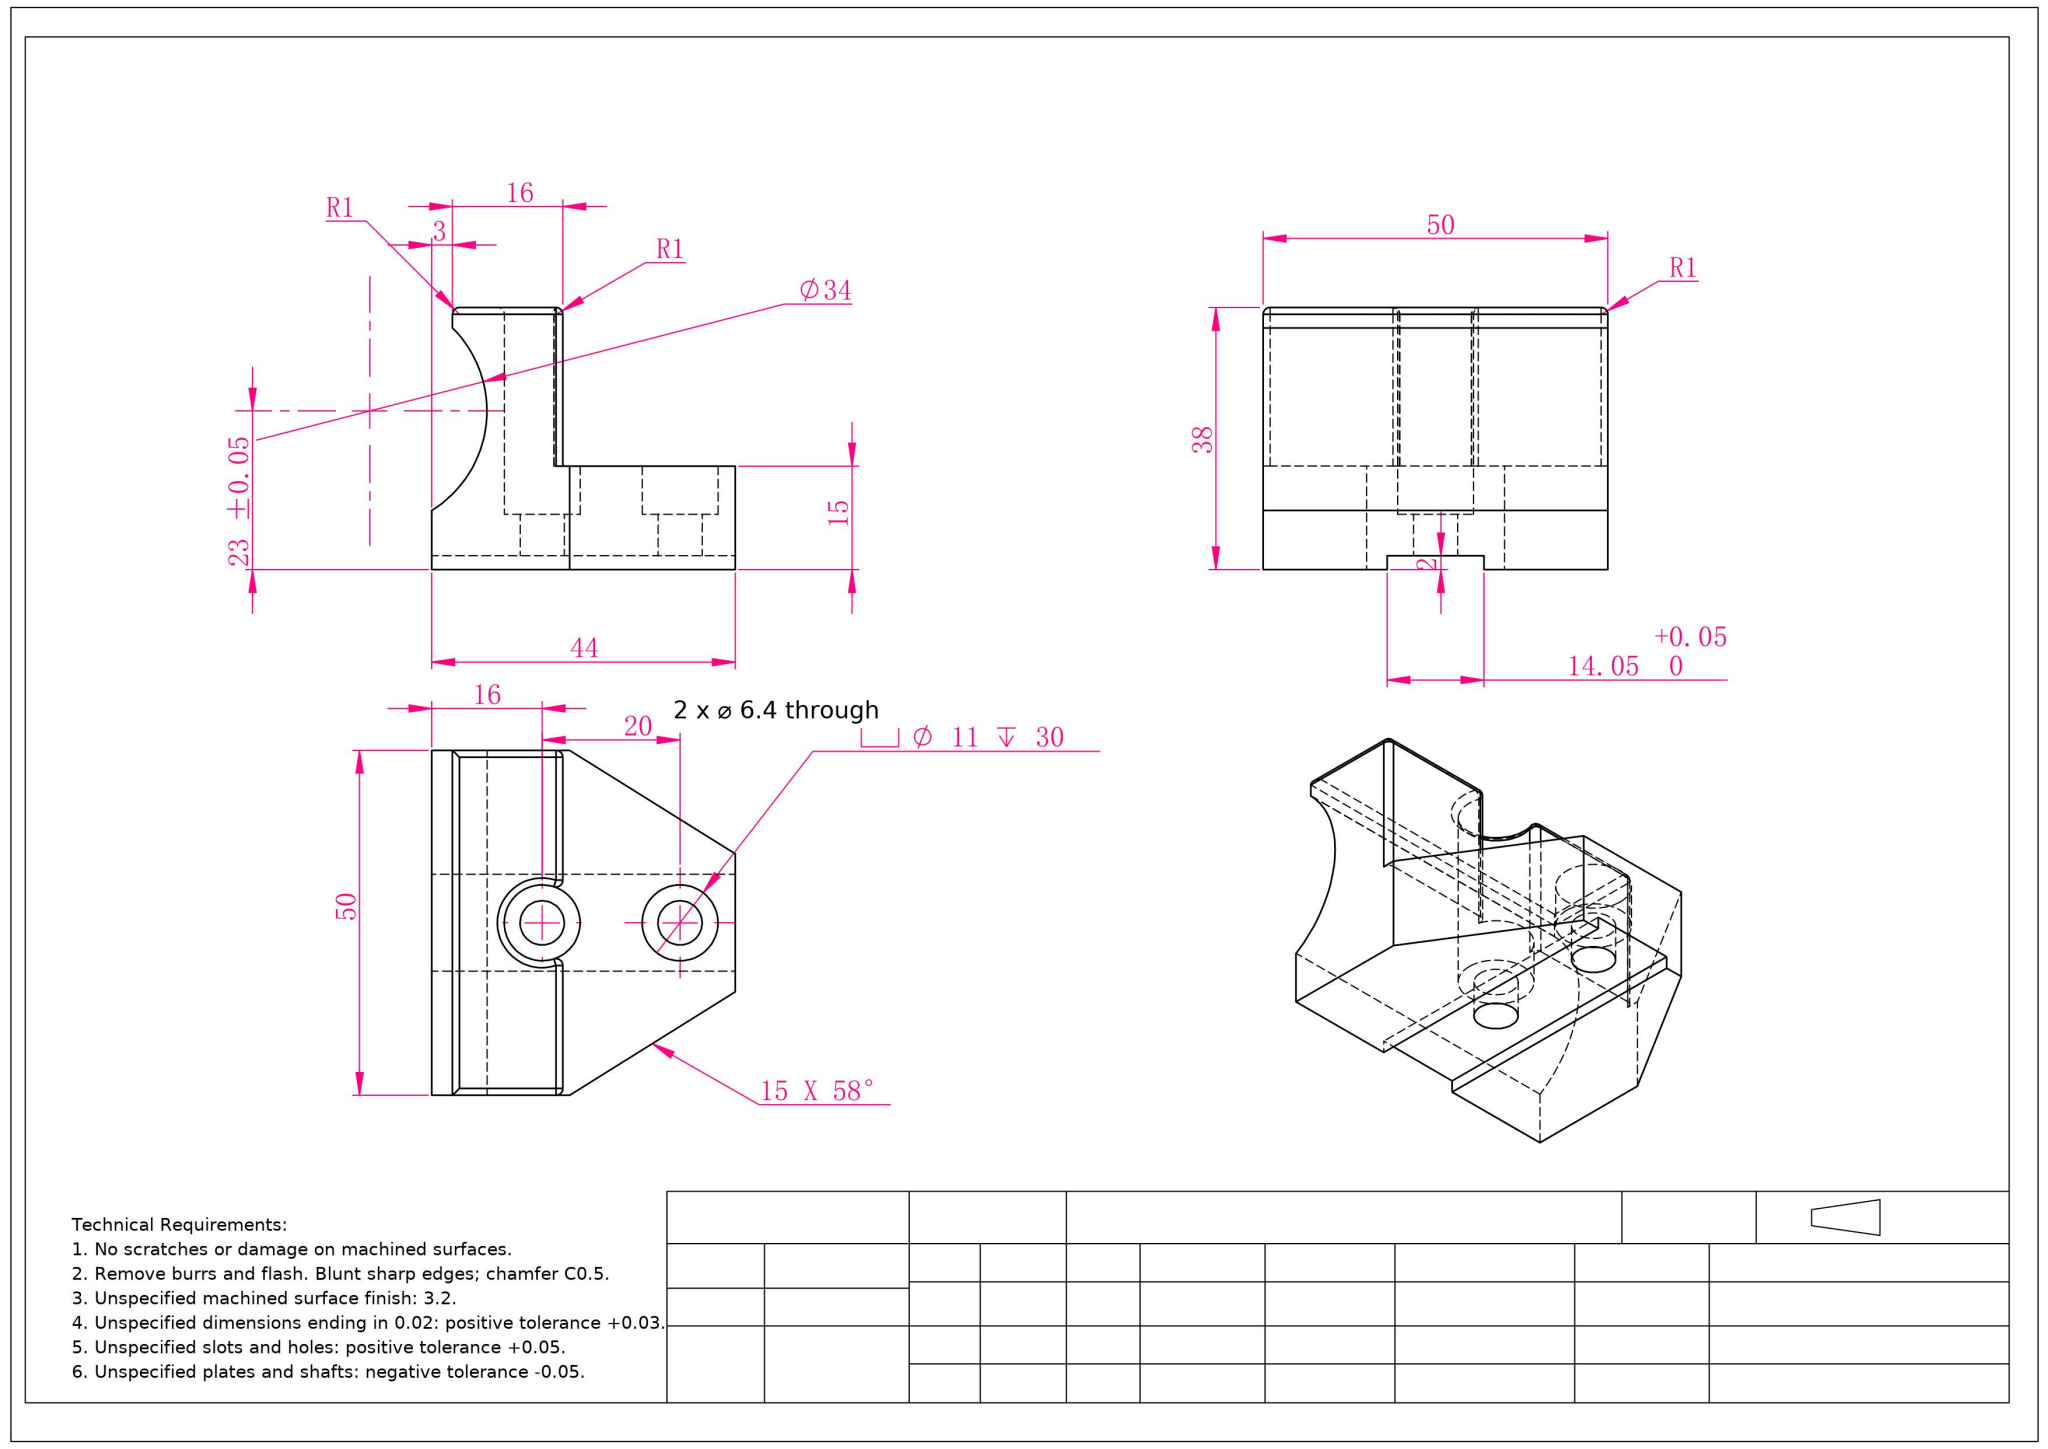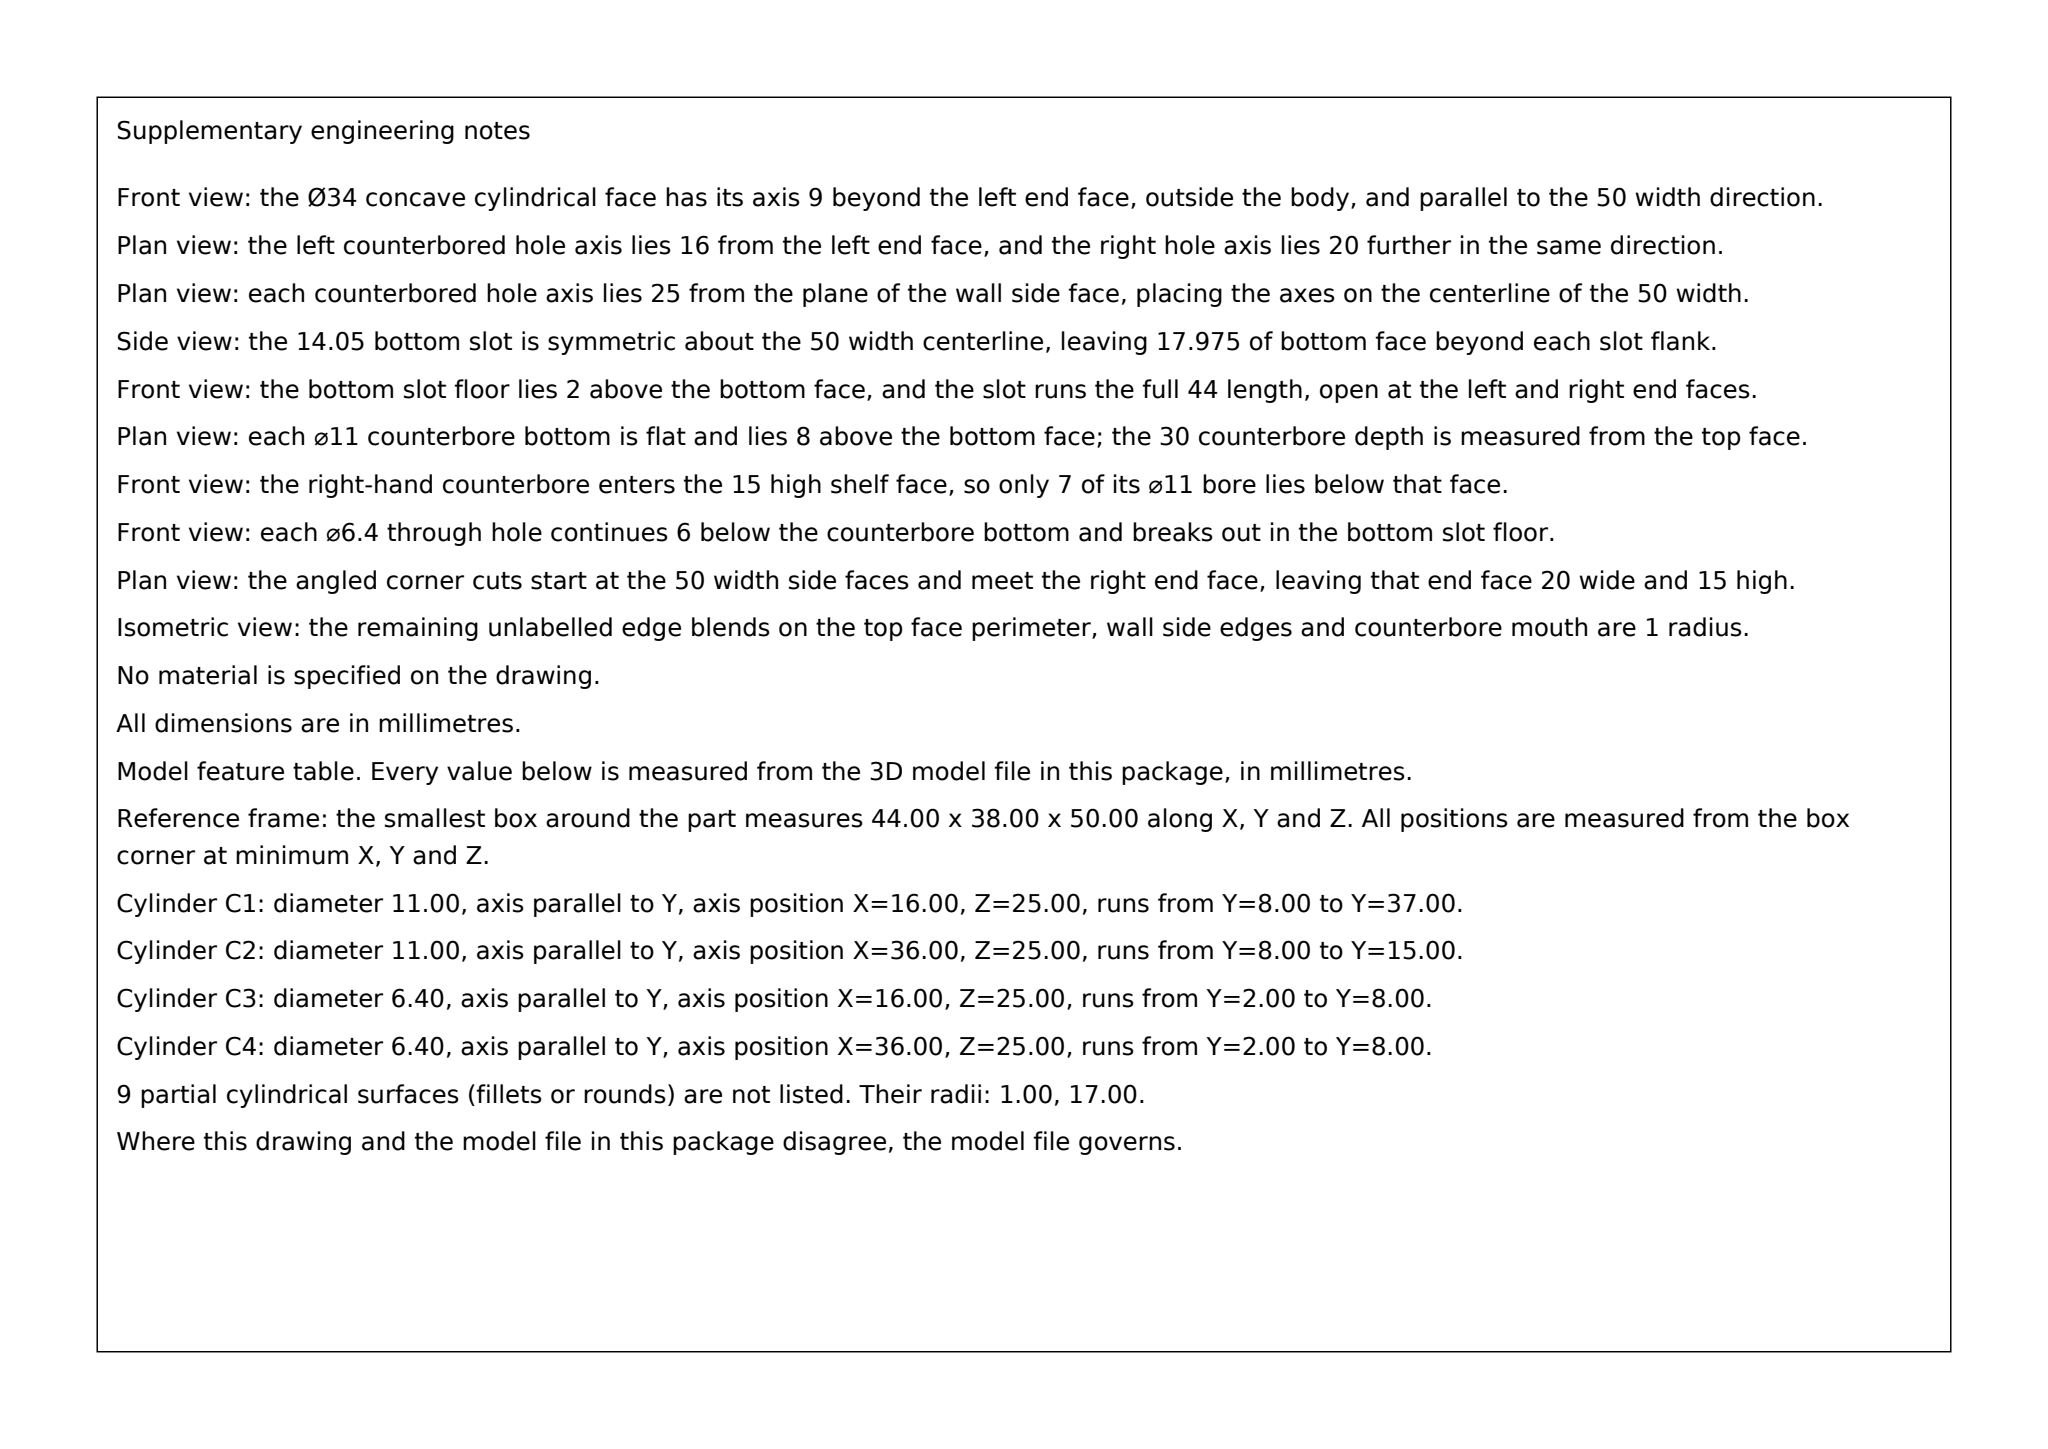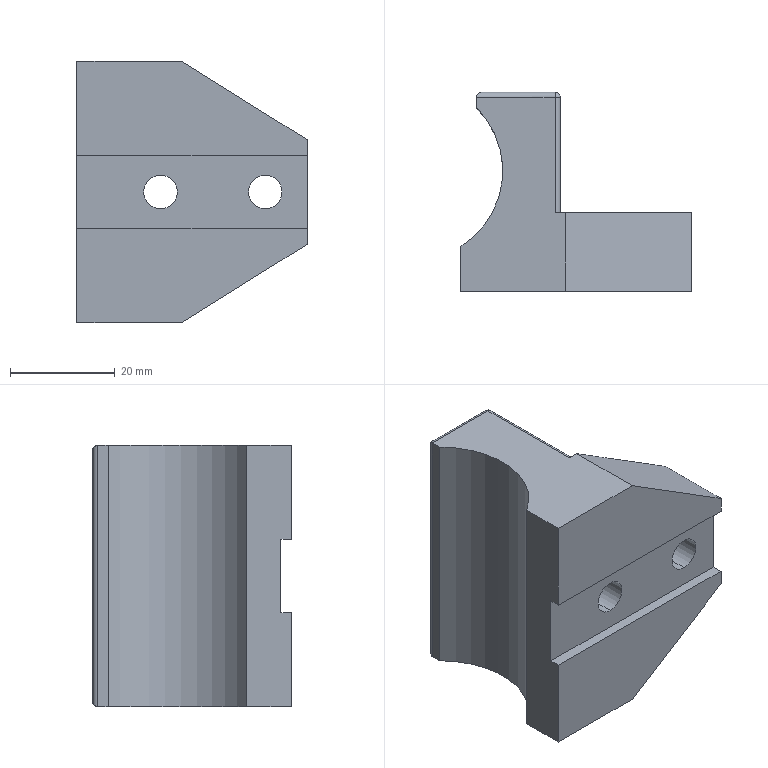Part | SolidWorks | mm | 1 solid | 44 faces | box 44 x 38 x 50 mm | volume 36222 mm3 | cylinder 19 | plane 18 | sphere 4 | torus 3 | commonest cylinder face diameters 2 x10 11 x4 6.4 x4 34 x1
Drawing notes:
3 & 16 WALLS 50 DEEP; TOP NOTCH 14.36 W CL ON 50 CL | from the solid: R1 edge cyl at (4,37) axis z len 50; top edge cyls at (18,37) len 17.82, vert R1 at z=18.82 & 31.18 -> gap 17.82-32.18 (14.36) centred on z=25
Ø34 CUT-OUT CL 9 OUTSIDE LH FACE, 23±0.05 UP FROM BASE | from the solid: cyl dia34 axis z at (x=-9, y=23); bbox x-min face x=0, base y=0
BOT SLOT 14.05 +0.05/0 W x 2 DP, 17.98 FROM FRONT 50 FACE | from the solid: z planes 17.98 & 32.03 (14.05 apart); y plane 2.0 = slot depth from y=0
2X Ø6.4 CBORE: 1ST CL 16 FROM LH FACE, 20 CTC, ON 50 CL | from the solid: dia6.4 axes y at x=16 and x=36, both z=25 (=50/2); spacing 20
NOTCH IN WALL BACK FACE: 14.36 W x 2 DP, 23 DOWN FROM TOP TO BASE | from the solid: R1 vert fillets at x=18, z=18.82/31.18 (len 22, y=15..37) => slot 17.82-32.18 (14.36 W, CL 25); fillet tangent x=17 vs back face x=19 (plane x=19 count 2) => 2 deep; wall y=15..38 => 23 from top face
HOLE AT 20 CTC: C'BORE Ø11 DP 7 FROM 15 BASE TOP FACE | from the solid: cylinder [11.0,"y",[36,null,25],7] vs [11.0,"y",[16,null,25],29]; base top plane y=15
build123d program:
from build123d import *
from OCP.BRepFilletAPI import BRepFilletAPI_MakeChamfer

# Parameters (mm, degrees)
BOSS_EXTRUDE1_DEPTH                             = 25
SKETCH2_W                                       = 45
SKETCH2_H                                       = 14.05
CUT_EXTRUDE1_DEPTH                              = 2
M6_HEX_SOCKET_HEAD_CAP_SCREW_CBORE1_D           = 6.4
M6_HEX_SOCKET_HEAD_CAP_SCREW_CBORE1_CBORE_D     = 11
M6_HEX_SOCKET_HEAD_CAP_SCREW_CBORE1_CBORE_DEPTH = 30
SKETCH6_W                                       = 25
SKETCH6_H                                       = 23
CUT_EXTRUDE3_DEPTH                              = 67.71
CUT_EXTRUDE4_DEPTH                              = 67.71
CHAMFER1_SIZE                                   = 15
CHAMFER1_SIZE2                                  = 24.005
FILLET1_R                                       = 1


with BuildPart() as part:
    # Sketch1 → Boss-Extrude1 (new, symmetric)
    with BuildSketch(Plane.XY):
        with BuildLine():
            Line((-22.5, 8), (-22.5, 0))
            Line((-22.5, 0), (22.5, 0))
            Line((22.5, 0), (22.5, 38))
            Line((22.5, 38), (-22.5, 38))
            ThreePointArc((-22.5, 38), (-15.923, 31.746), (-13.5, 23))
            ThreePointArc((-13.5, 23), (-15.923, 14.254), (-22.5, 8))
        make_face()
    extrude(amount=BOSS_EXTRUDE1_DEPTH, both=True)

    # Sketch2 → Cut-Extrude1 (cut)
    with BuildSketch(Plane.XZ):
        Rectangle(SKETCH2_W, SKETCH2_H)
    extrude(amount=-CUT_EXTRUDE1_DEPTH, mode=Mode.SUBTRACT)

    # M6 Hex Socket Head Cap Screw CBORE1 (through all)
    with Locations(Plane(origin=(0, 38, 0), x_dir=(1, 0, 0), z_dir=(0, 1, 0))):
        with Locations((-5.5, 0), (14.5, 0)):
            CounterBoreHole(M6_HEX_SOCKET_HEAD_CAP_SCREW_CBORE1_D / 2, M6_HEX_SOCKET_HEAD_CAP_SCREW_CBORE1_CBORE_D / 2, M6_HEX_SOCKET_HEAD_CAP_SCREW_CBORE1_CBORE_DEPTH)

    # Sketch6 → Cut-Extrude3 (cut, through all)
    with BuildSketch(Plane(origin=(0, 0, -25), x_dir=(-1, 0, 0), z_dir=(0, 0, -1))):
        with Locations((-10, 26.5)):
            Rectangle(SKETCH6_W, SKETCH6_H)
    extrude(amount=-CUT_EXTRUDE3_DEPTH, mode=Mode.SUBTRACT)

    # Sketch8 → Cut-Extrude4 (cut, through all)
    with BuildSketch(Plane(origin=(0, 0, -25), x_dir=(-1, 0, 0), z_dir=(0, 0, -1))):
        Polygon((18.5, 38), (18.5, 20), (21.5, 20), (21.5, 0), (41.306, 0), (41.306, 38), align=None)
    extrude(amount=-CUT_EXTRUDE4_DEPTH, mode=Mode.SUBTRACT)

    # Chamfer1: one chamfer whose edges measure the first distance from different faces: ONE call of the kernel's chamfer builder (chamfer() names one face for all edges)
    chamfer1_edges_1 = [part.edges().sort_by_distance(p)[0] for p in [
        (22.5, 7.5, -25),
    ]]
    chamfer1_side_1 = [part.faces().sort_by_distance(p)[0] for p in [
        (22.5, 7.753, -12.85),
    ]]
    chamfer1_edges_2 = [part.edges().sort_by_distance(p)[0] for p in [
        (22.5, 7.5, 25),
    ]]
    chamfer1_side_2 = [part.faces().sort_by_distance(p)[0] for p in [
        (22.5, 7.753, 12.85),
    ]]
    chamfer1 = BRepFilletAPI_MakeChamfer(part.part.solid().wrapped)
    for e in chamfer1_edges_1:
        chamfer1.Add(CHAMFER1_SIZE, CHAMFER1_SIZE2, e.wrapped, chamfer1_side_1[0].wrapped)  # the first distance lies on this face
    for e in chamfer1_edges_2:
        chamfer1.Add(CHAMFER1_SIZE, CHAMFER1_SIZE2, e.wrapped, chamfer1_side_2[0].wrapped)  # the first distance lies on this face
    add(Compound.cast(chamfer1.Shape()), mode=Mode.REPLACE)

    # Fillet1
    fillet1_edges = [part.edges().sort_by_distance(p)[0] for p in [
        (-11, 38, 0),
        (-2.5, 26.5, -4.61),
        (-2.5, 26.5, 4.61),
        (-2.5, 38, 14.805),
        (-2.5, 26.5, 25),
        (-2.5, 38, -14.805),
        (-2.5, 26.5, -25),
        (-10.5, 38, -25),
        (-10.5, 38, 25),
        (-18.5, 38, 0),
    ]]
    fillet(fillet1_edges, radius=FILLET1_R)


solid = part.part